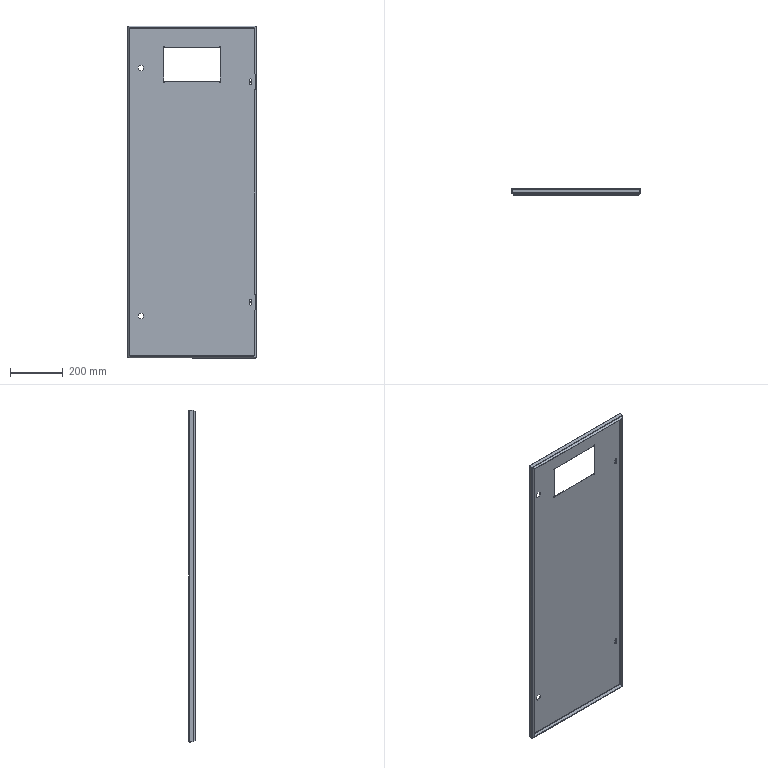Component | SolidWorks | 500CabinetWidthLowerDoor-1 | 1 solid | 122 faces | volume 1012245 mm3 | plane 72 | cylinder 34 | spline 16 | commonest cylinder face diameters 5 x10 2 x10 9.5 x8 5.5 x6 | material Plain Carbon Steel